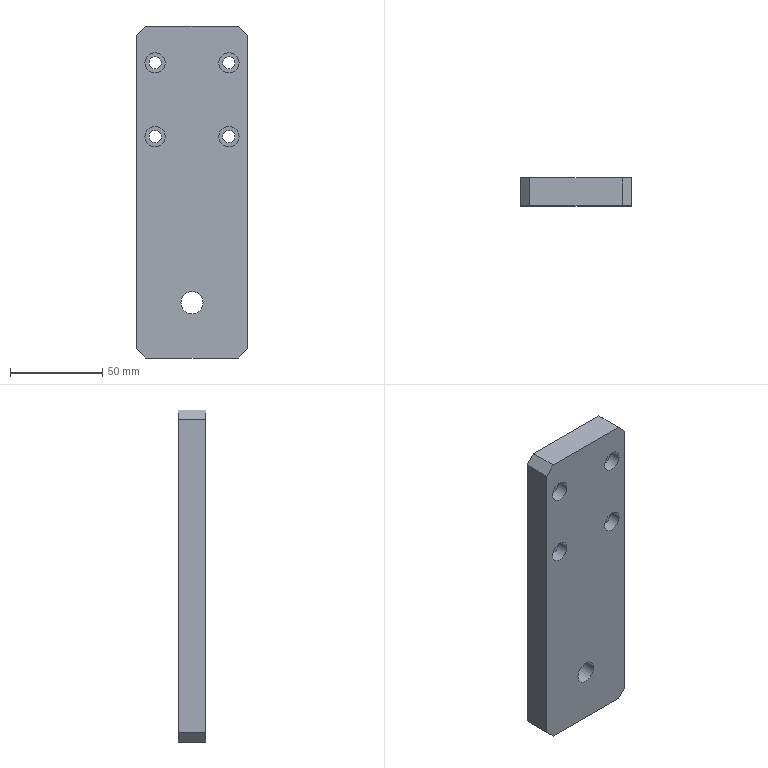Component | SolidWorks | 8TC-A15004-80-15A-5 | 1 solid | 32 faces | box 60 x 15 x 180 mm | volume 155944 mm3 | cylinder 18 | plane 14 | commonest cylinder face diameters 11 x8 6.6 x8 12 x2 | material A3
build123d program:
from build123d import *

# Parameters (mm, degrees)
SKETCH1_W                                       = 180
SKETCH1_H                                       = 60
BOSS_EXTRUDE1_DEPTH                             = 7.5
SKETCH2_R                                       = 6
CUT_EXTRUDE1_DEPTH                              = 97.047
CHAMFER1_SIZE                                   = 5
M6_HEX_SOCKET_HEAD_CAP_SCREW_CBORE1_D           = 6.6
M6_HEX_SOCKET_HEAD_CAP_SCREW_CBORE1_CBORE_D     = 11
M6_HEX_SOCKET_HEAD_CAP_SCREW_CBORE1_CBORE_DEPTH = 6.4


with BuildPart() as part:
    # Sketch1 → Boss-Extrude1 (new, symmetric)
    with BuildSketch(Plane(origin=(0, 0, 0), x_dir=(1, 0, 0), z_dir=(0, 1, 0))):
        Rectangle(SKETCH1_W, SKETCH1_H)
    extrude(amount=BOSS_EXTRUDE1_DEPTH, both=True)

    # Sketch2 → Cut-Extrude1 (cut, through all)
    with BuildSketch(Plane(origin=(0, 7.5, 0), x_dir=(1, 0, 0), z_dir=(0, 1, 0))):
        with Locations(Location((60, 0, 0), (0, 0, 270))):
            Circle(SKETCH2_R)
    extrude(amount=-CUT_EXTRUDE1_DEPTH, mode=Mode.SUBTRACT)

    # Chamfer1
    chamfer1_edges = [part.edges().sort_by_distance(p)[0] for p in [
        (90, 0, 30),
        (-90, 0, 30),
        (-90, 0, -30),
        (90, 0, -30),
    ]]
    chamfer(chamfer1_edges, length=CHAMFER1_SIZE)

    # M6 Hex Socket Head Cap Screw CBORE1 (through all)
    with Locations(Plane(origin=(0, 7.5, 0), x_dir=(1, 0, 0), z_dir=(0, 1, 0))):
        with Locations((-70, 20), (-30, 20), (-30, -20), (-70, -20)):
            CounterBoreHole(M6_HEX_SOCKET_HEAD_CAP_SCREW_CBORE1_D / 2, M6_HEX_SOCKET_HEAD_CAP_SCREW_CBORE1_CBORE_D / 2, M6_HEX_SOCKET_HEAD_CAP_SCREW_CBORE1_CBORE_DEPTH)


solid = part.part

# Placed as in the assembly
solid = solid.moved(Location((40, -15, -690), (180, -90, 0)))
STEP:
#1=CARTESIAN_POINT('',(2.579,-0.6339,-24.409));
#2=VERTEX_POINT('',#1);
#3=CARTESIAN_POINT('',(2.146,-0.6339,-24.409));
#4=VERTEX_POINT('',#3);
#5=CARTESIAN_POINT('',(2.362,-0.6339,-24.409));
#6=DIRECTION('',(0.,-1.,0.));
#7=DIRECTION('',(-1.,0.,0.));
#8=AXIS2_PLACEMENT_3D('',#5,#6,#7);
#9=CIRCLE('',#8,0.2165);
#10=EDGE_CURVE('',#2,#4,#9,.T.);
#11=ORIENTED_EDGE('',*,*,#10,.F.);
#12=CARTESIAN_POINT('',(2.579,-0.8858,-24.409));
#13=VERTEX_POINT('',#12);
#14=CARTESIAN_POINT('',(2.579,-0.8858,-24.409));
#15=DIRECTION('',(0.,-1.,0.));
#16=VECTOR('',#15,39.37);
#17=LINE('',#14,#16);
#18=EDGE_CURVE('',#2,#13,#17,.T.);
#19=ORIENTED_EDGE('',*,*,#18,.T.);
#20=CARTESIAN_POINT('',(2.146,-0.8858,-24.409));
#21=VERTEX_POINT('',#20);
#22=CARTESIAN_POINT('',(2.362,-0.8858,-24.409));
#23=DIRECTION('',(0.,-1.,0.));
#24=DIRECTION('',(-1.,0.,0.));
#25=AXIS2_PLACEMENT_3D('',#22,#23,#24);
#26=CIRCLE('',#25,0.2165);
#27=EDGE_CURVE('',#13,#21,#26,.T.);
#28=ORIENTED_EDGE('',*,*,#27,.T.);
#29=CARTESIAN_POINT('',(2.146,-0.8858,-24.409));
#30=DIRECTION('',(0.,-1.,0.));
#31=VECTOR('',#30,39.37);
#32=LINE('',#29,#31);
#33=EDGE_CURVE('',#4,#21,#32,.T.);
#34=ORIENTED_EDGE('',*,*,#33,.F.);
#35=EDGE_LOOP('',(#11,#19,#28,#34));
#36=FACE_OUTER_BOUND('',#35,.T.);
#37=CARTESIAN_POINT('',(2.362,-0.8858,-24.409));
#38=DIRECTION('',(0.,-1.,0.));
#39=DIRECTION('',(-1.,0.,0.));
#40=AXIS2_PLACEMENT_3D('',#37,#38,#39);
#41=CYLINDRICAL_SURFACE('',#40,0.2165);
#42=ADVANCED_FACE('',(#36),#41,.F.);
#43=CARTESIAN_POINT('',(2.492,-0.2953,-24.409));
#44=VERTEX_POINT('',#43);
#45=CARTESIAN_POINT('',(2.232,-0.2953,-24.409));
#46=VERTEX_POINT('',#45);
#47=CARTESIAN_POINT('',(2.362,-0.2953,-24.409));
#48=DIRECTION('',(0.,-1.,0.));
#49=DIRECTION('',(-1.,0.,0.));
#50=AXIS2_PLACEMENT_3D('',#47,#48,#49);
#51=CIRCLE('',#50,0.1299);
#52=EDGE_CURVE('',#44,#46,#51,.T.);
#53=ORIENTED_EDGE('',*,*,#52,.F.);
#54=CARTESIAN_POINT('',(2.492,-0.6339,-24.409));
#55=VERTEX_POINT('',#54);
#56=CARTESIAN_POINT('',(2.492,-0.8858,-24.409));
#57=DIRECTION('',(0.,-1.,0.));
#58=VECTOR('',#57,39.37);
#59=LINE('',#56,#58);
#60=EDGE_CURVE('',#44,#55,#59,.T.);
#61=ORIENTED_EDGE('',*,*,#60,.T.);
#62=CARTESIAN_POINT('',(2.232,-0.6339,-24.409));
#63=VERTEX_POINT('',#62);
#64=CARTESIAN_POINT('',(2.362,-0.6339,-24.409));
#65=DIRECTION('',(0.,-1.,0.));
#66=DIRECTION('',(-1.,0.,0.));
#67=AXIS2_PLACEMENT_3D('',#64,#65,#66);
#68=CIRCLE('',#67,0.1299);
#69=EDGE_CURVE('',#55,#63,#68,.T.);
#70=ORIENTED_EDGE('',*,*,#69,.T.);
#71=CARTESIAN_POINT('',(2.232,-0.8858,-24.409));
#72=DIRECTION('',(0.,-1.,0.));
#73=VECTOR('',#72,39.37);
#74=LINE('',#71,#73);
#75=EDGE_CURVE('',#46,#63,#74,.T.);
#76=ORIENTED_EDGE('',*,*,#75,.F.);
#77=EDGE_LOOP('',(#53,#61,#70,#76));
#78=FACE_OUTER_BOUND('',#77,.T.);
#79=CARTESIAN_POINT('',(2.362,-0.8858,-24.409));
#80=DIRECTION('',(0.,-1.,0.));
#81=DIRECTION('',(-1.,0.,0.));
#82=AXIS2_PLACEMENT_3D('',#79,#80,#81);
#83=CYLINDRICAL_SURFACE('',#82,0.1299);
#84=ADVANCED_FACE('',(#78),#83,.F.);
#85=CARTESIAN_POINT('',(2.579,-0.6339,-25.984));
#86=VERTEX_POINT('',#85);
#87=CARTESIAN_POINT('',(2.146,-0.6339,-25.984));
#88=VERTEX_POINT('',#87);
#89=CARTESIAN_POINT('',(2.362,-0.6339,-25.984));
#90=DIRECTION('',(0.,-1.,0.));
#91=DIRECTION('',(-1.,0.,0.));
#92=AXIS2_PLACEMENT_3D('',#89,#90,#91);
#93=CIRCLE('',#92,0.2165);
#94=EDGE_CURVE('',#86,#88,#93,.T.);
#95=ORIENTED_EDGE('',*,*,#94,.F.);
#96=CARTESIAN_POINT('',(2.579,-0.8858,-25.984));
#97=VERTEX_POINT('',#96);
#98=CARTESIAN_POINT('',(2.579,-0.8858,-25.984));
#99=DIRECTION('',(0.,-1.,0.));
#100=VECTOR('',#99,39.37);
#101=LINE('',#98,#100);
#102=EDGE_CURVE('',#86,#97,#101,.T.);
#103=ORIENTED_EDGE('',*,*,#102,.T.);
#104=CARTESIAN_POINT('',(2.146,-0.8858,-25.984));
#105=VERTEX_POINT('',#104);
#106=CARTESIAN_POINT('',(2.362,-0.8858,-25.984));
#107=DIRECTION('',(0.,-1.,0.));
#108=DIRECTION('',(-1.,0.,0.));
#109=AXIS2_PLACEMENT_3D('',#106,#107,#108);
#110=CIRCLE('',#109,0.2165);
#111=EDGE_CURVE('',#97,#105,#110,.T.);
#112=ORIENTED_EDGE('',*,*,#111,.T.);
#113=CARTESIAN_POINT('',(2.146,-0.8858,-25.984));
#114=DIRECTION('',(0.,-1.,0.));
#115=VECTOR('',#114,39.37);
#116=LINE('',#113,#115);
#117=EDGE_CURVE('',#88,#105,#116,.T.);
#118=ORIENTED_EDGE('',*,*,#117,.F.);
#119=EDGE_LOOP('',(#95,#103,#112,#118));
#120=FACE_OUTER_BOUND('',#119,.T.);
#121=CARTESIAN_POINT('',(2.362,-0.8858,-25.984));
#122=DIRECTION('',(0.,-1.,0.));
#123=DIRECTION('',(-1.,0.,0.));
#124=AXIS2_PLACEMENT_3D('',#121,#122,#123);
#125=CYLINDRICAL_SURFACE('',#124,0.2165);
#126=ADVANCED_FACE('',(#120),#125,.F.);
#127=CARTESIAN_POINT('',(2.492,-0.2953,-25.984));
#128=VERTEX_POINT('',#127);
#129=CARTESIAN_POINT('',(2.232,-0.2953,-25.984));
#130=VERTEX_POINT('',#129);
#131=CARTESIAN_POINT('',(2.362,-0.2953,-25.984));
#132=DIRECTION('',(0.,-1.,0.));
#133=DIRECTION('',(-1.,0.,0.));
#134=AXIS2_PLACEMENT_3D('',#131,#132,#133);
#135=CIRCLE('',#134,0.1299);
#136=EDGE_CURVE('',#128,#130,#135,.T.);
#137=ORIENTED_EDGE('',*,*,#136,.F.);
#138=CARTESIAN_POINT('',(2.492,-0.6339,-25.984));
#139=VERTEX_POINT('',#138);
#140=CARTESIAN_POINT('',(2.492,-0.8858,-25.984));
#141=DIRECTION('',(0.,-1.,0.));
#142=VECTOR('',#141,39.37);
#143=LINE('',#140,#142);
#144=EDGE_CURVE('',#128,#139,#143,.T.);
#145=ORIENTED_EDGE('',*,*,#144,.T.);
#146=CARTESIAN_POINT('',(2.232,-0.6339,-25.984));
#147=VERTEX_POINT('',#146);
#148=CARTESIAN_POINT('',(2.362,-0.6339,-25.984));
#149=DIRECTION('',(0.,-1.,0.));
#150=DIRECTION('',(-1.,0.,0.));
#151=AXIS2_PLACEMENT_3D('',#148,#149,#150);
#152=CIRCLE('',#151,0.1299);
#153=EDGE_CURVE('',#139,#147,#152,.T.);
#154=ORIENTED_EDGE('',*,*,#153,.T.);
#155=CARTESIAN_POINT('',(2.232,-0.8858,-25.984));
#156=DIRECTION('',(0.,-1.,0.));
#157=VECTOR('',#156,39.37);
#158=LINE('',#155,#157);
#159=EDGE_CURVE('',#130,#147,#158,.T.);
#160=ORIENTED_EDGE('',*,*,#159,.F.);
#161=EDGE_LOOP('',(#137,#145,#154,#160));
#162=FACE_OUTER_BOUND('',#161,.T.);
#163=CARTESIAN_POINT('',(2.362,-0.8858,-25.984));
#164=DIRECTION('',(0.,-1.,0.));
#165=DIRECTION('',(-1.,0.,0.));
#166=AXIS2_PLACEMENT_3D('',#163,#164,#165);
#167=CYLINDRICAL_SURFACE('',#166,0.1299);
#168=ADVANCED_FACE('',(#162),#167,.F.);
#169=CARTESIAN_POINT('',(1.004,-0.6339,-25.984));
#170=VERTEX_POINT('',#169);
#171=CARTESIAN_POINT('',(0.5709,-0.6339,-25.984));
#172=VERTEX_POINT('',#171);
#173=CARTESIAN_POINT('',(0.7874,-0.6339,-25.984));
#174=DIRECTION('',(0.,-1.,0.));
#175=DIRECTION('',(-1.,0.,0.));
#176=AXIS2_PLACEMENT_3D('',#173,#174,#175);
#177=CIRCLE('',#176,0.2165);
#178=EDGE_CURVE('',#170,#172,#177,.T.);
#179=ORIENTED_EDGE('',*,*,#178,.F.);
#180=CARTESIAN_POINT('',(1.004,-0.8858,-25.984));
#181=VERTEX_POINT('',#180);
#182=CARTESIAN_POINT('',(1.004,-0.8858,-25.984));
#183=DIRECTION('',(0.,-1.,0.));
#184=VECTOR('',#183,39.37);
#185=LINE('',#182,#184);
#186=EDGE_CURVE('',#170,#181,#185,.T.);
#187=ORIENTED_EDGE('',*,*,#186,.T.);
#188=CARTESIAN_POINT('',(0.5709,-0.8858,-25.984));
#189=VERTEX_POINT('',#188);
#190=CARTESIAN_POINT('',(0.7874,-0.8858,-25.984));
#191=DIRECTION('',(0.,-1.,0.));
#192=DIRECTION('',(-1.,0.,0.));
#193=AXIS2_PLACEMENT_3D('',#190,#191,#192);
#194=CIRCLE('',#193,0.2165);
#195=EDGE_CURVE('',#181,#189,#194,.T.);
#196=ORIENTED_EDGE('',*,*,#195,.T.);
#197=CARTESIAN_POINT('',(0.5709,-0.8858,-25.984));
#198=DIRECTION('',(0.,-1.,0.));
#199=VECTOR('',#198,39.37);
#200=LINE('',#197,#199);
#201=EDGE_CURVE('',#172,#189,#200,.T.);
#202=ORIENTED_EDGE('',*,*,#201,.F.);
#203=EDGE_LOOP('',(#179,#187,#196,#202));
#204=FACE_OUTER_BOUND('',#203,.T.);
#205=CARTESIAN_POINT('',(0.7874,-0.8858,-25.984));
#206=DIRECTION('',(0.,-1.,0.));
#207=DIRECTION('',(-1.,0.,0.));
#208=AXIS2_PLACEMENT_3D('',#205,#206,#207);
#209=CYLINDRICAL_SURFACE('',#208,0.2165);
#210=ADVANCED_FACE('',(#204),#209,.F.);
#211=CARTESIAN_POINT('',(0.9173,-0.2953,-25.984));
#212=VERTEX_POINT('',#211);
#213=CARTESIAN_POINT('',(0.6575,-0.2953,-25.984));
#214=VERTEX_POINT('',#213);
#215=CARTESIAN_POINT('',(0.7874,-0.2953,-25.984));
#216=DIRECTION('',(0.,-1.,0.));
#217=DIRECTION('',(-1.,0.,0.));
#218=AXIS2_PLACEMENT_3D('',#215,#216,#217);
#219=CIRCLE('',#218,0.1299);
#220=EDGE_CURVE('',#212,#214,#219,.T.);
#221=ORIENTED_EDGE('',*,*,#220,.F.);
#222=CARTESIAN_POINT('',(0.9173,-0.6339,-25.984));
#223=VERTEX_POINT('',#222);
#224=CARTESIAN_POINT('',(0.9173,-0.8858,-25.984));
#225=DIRECTION('',(0.,-1.,0.));
#226=VECTOR('',#225,39.37);
#227=LINE('',#224,#226);
#228=EDGE_CURVE('',#212,#223,#227,.T.);
#229=ORIENTED_EDGE('',*,*,#228,.T.);
#230=CARTESIAN_POINT('',(0.6575,-0.6339,-25.984));
#231=VERTEX_POINT('',#230);
#232=CARTESIAN_POINT('',(0.7874,-0.6339,-25.984));
#233=DIRECTION('',(0.,-1.,0.));
#234=DIRECTION('',(-1.,0.,0.));
#235=AXIS2_PLACEMENT_3D('',#232,#233,#234);
#236=CIRCLE('',#235,0.1299);
#237=EDGE_CURVE('',#223,#231,#236,.T.);
#238=ORIENTED_EDGE('',*,*,#237,.T.);
#239=CARTESIAN_POINT('',(0.6575,-0.8858,-25.984));
#240=DIRECTION('',(0.,-1.,0.));
#241=VECTOR('',#240,39.37);
#242=LINE('',#239,#241);
#243=EDGE_CURVE('',#214,#231,#242,.T.);
#244=ORIENTED_EDGE('',*,*,#243,.F.);
#245=EDGE_LOOP('',(#221,#229,#238,#244));
#246=FACE_OUTER_BOUND('',#245,.T.);
#247=CARTESIAN_POINT('',(0.7874,-0.8858,-25.984));
#248=DIRECTION('',(0.,-1.,0.));
#249=DIRECTION('',(-1.,0.,0.));
#250=AXIS2_PLACEMENT_3D('',#247,#248,#249);
#251=CYLINDRICAL_SURFACE('',#250,0.1299);
#252=ADVANCED_FACE('',(#246),#251,.F.);
#253=CARTESIAN_POINT('',(1.004,-0.6339,-24.409));
#254=VERTEX_POINT('',#253);
#255=CARTESIAN_POINT('',(0.5709,-0.6339,-24.409));
#256=VERTEX_POINT('',#255);
#257=CARTESIAN_POINT('',(0.7874,-0.6339,-24.409));
#258=DIRECTION('',(0.,-1.,0.));
#259=DIRECTION('',(-1.,0.,0.));
#260=AXIS2_PLACEMENT_3D('',#257,#258,#259);
#261=CIRCLE('',#260,0.2165);
#262=EDGE_CURVE('',#254,#256,#261,.T.);
#263=ORIENTED_EDGE('',*,*,#262,.F.);
#264=CARTESIAN_POINT('',(1.004,-0.8858,-24.409));
#265=VERTEX_POINT('',#264);
#266=CARTESIAN_POINT('',(1.004,-0.8858,-24.409));
#267=DIRECTION('',(0.,-1.,0.));
#268=VECTOR('',#267,39.37);
#269=LINE('',#266,#268);
#270=EDGE_CURVE('',#254,#265,#269,.T.);
#271=ORIENTED_EDGE('',*,*,#270,.T.);
#272=CARTESIAN_POINT('',(0.5709,-0.8858,-24.409));
#273=VERTEX_POINT('',#272);
#274=CARTESIAN_POINT('',(0.7874,-0.8858,-24.409));
#275=DIRECTION('',(0.,-1.,0.));
#276=DIRECTION('',(-1.,0.,0.));
#277=AXIS2_PLACEMENT_3D('',#274,#275,#276);
#278=CIRCLE('',#277,0.2165);
#279=EDGE_CURVE('',#265,#273,#278,.T.);
#280=ORIENTED_EDGE('',*,*,#279,.T.);
#281=CARTESIAN_POINT('',(0.5709,-0.8858,-24.409));
#282=DIRECTION('',(0.,-1.,0.));
#283=VECTOR('',#282,39.37);
#284=LINE('',#281,#283);
#285=EDGE_CURVE('',#256,#273,#284,.T.);
#286=ORIENTED_EDGE('',*,*,#285,.F.);
#287=EDGE_LOOP('',(#263,#271,#280,#286));
#288=FACE_OUTER_BOUND('',#287,.T.);
#289=CARTESIAN_POINT('',(0.7874,-0.8858,-24.409));
#290=DIRECTION('',(0.,-1.,0.));
#291=DIRECTION('',(-1.,0.,0.));
#292=AXIS2_PLACEMENT_3D('',#289,#290,#291);
#293=CYLINDRICAL_SURFACE('',#292,0.2165);
#294=ADVANCED_FACE('',(#288),#293,.F.);
#295=CARTESIAN_POINT('',(0.9173,-0.2953,-24.409));
#296=VERTEX_POINT('',#295);
#297=CARTESIAN_POINT('',(0.6575,-0.2953,-24.409));
#298=VERTEX_POINT('',#297);
#299=CARTESIAN_POINT('',(0.7874,-0.2953,-24.409));
#300=DIRECTION('',(0.,-1.,0.));
#301=DIRECTION('',(-1.,0.,0.));
#302=AXIS2_PLACEMENT_3D('',#299,#300,#301);
#303=CIRCLE('',#302,0.1299);
#304=EDGE_CURVE('',#296,#298,#303,.T.);
#305=ORIENTED_EDGE('',*,*,#304,.F.);
#306=CARTESIAN_POINT('',(0.9173,-0.6339,-24.409));
#307=VERTEX_POINT('',#306);
#308=CARTESIAN_POINT('',(0.9173,-0.8858,-24.409));
#309=DIRECTION('',(0.,-1.,0.));
#310=VECTOR('',#309,39.37);
#311=LINE('',#308,#310);
#312=EDGE_CURVE('',#296,#307,#311,.T.);
#313=ORIENTED_EDGE('',*,*,#312,.T.);
#314=CARTESIAN_POINT('',(0.6575,-0.6339,-24.409));
#315=VERTEX_POINT('',#314);
#316=CARTESIAN_POINT('',(0.7874,-0.6339,-24.409));
#317=DIRECTION('',(0.,-1.,0.));
#318=DIRECTION('',(-1.,0.,0.));
#319=AXIS2_PLACEMENT_3D('',#316,#317,#318);
#320=CIRCLE('',#319,0.1299);
#321=EDGE_CURVE('',#307,#315,#320,.T.);
#322=ORIENTED_EDGE('',*,*,#321,.T.);
#323=CARTESIAN_POINT('',(0.6575,-0.8858,-24.409));
#324=DIRECTION('',(0.,-1.,0.));
#325=VECTOR('',#324,39.37);
#326=LINE('',#323,#325);
#327=EDGE_CURVE('',#298,#315,#326,.T.);
#328=ORIENTED_EDGE('',*,*,#327,.F.);
#329=EDGE_LOOP('',(#305,#313,#322,#328));
#330=FACE_OUTER_BOUND('',#329,.T.);
#331=CARTESIAN_POINT('',(0.7874,-0.8858,-24.409));
#332=DIRECTION('',(0.,-1.,0.));
#333=DIRECTION('',(-1.,0.,0.));
#334=AXIS2_PLACEMENT_3D('',#331,#332,#333);
#335=CYLINDRICAL_SURFACE('',#334,0.1299);
#336=ADVANCED_FACE('',(#330),#335,.F.);
#337=CARTESIAN_POINT('',(1.811,-0.2953,-29.528));
#338=VERTEX_POINT('',#337);
#339=CARTESIAN_POINT('',(1.339,-0.2953,-29.528));
#340=VERTEX_POINT('',#339);
#341=CARTESIAN_POINT('',(1.575,-0.2953,-29.528));
#342=DIRECTION('',(0.,-1.,0.));
#343=DIRECTION('',(-1.,0.,0.));
#344=AXIS2_PLACEMENT_3D('',#341,#342,#343);
#345=CIRCLE('',#344,0.2362);
#346=EDGE_CURVE('',#338,#340,#345,.T.);
#347=ORIENTED_EDGE('',*,*,#346,.F.);
#348=CARTESIAN_POINT('',(1.811,-0.8858,-29.528));
#349=VERTEX_POINT('',#348);
#350=CARTESIAN_POINT('',(1.811,-0.2953,-29.528));
#351=DIRECTION('',(0.,-1.,0.));
#352=VECTOR('',#351,39.37);
#353=LINE('',#350,#352);
#354=EDGE_CURVE('',#338,#349,#353,.T.);
#355=ORIENTED_EDGE('',*,*,#354,.T.);
#356=CARTESIAN_POINT('',(1.339,-0.8858,-29.528));
#357=VERTEX_POINT('',#356);
#358=CARTESIAN_POINT('',(1.575,-0.8858,-29.528));
#359=DIRECTION('',(0.,-1.,0.));
#360=DIRECTION('',(-1.,0.,0.));
#361=AXIS2_PLACEMENT_3D('',#358,#359,#360);
#362=CIRCLE('',#361,0.2362);
#363=EDGE_CURVE('',#349,#357,#362,.T.);
#364=ORIENTED_EDGE('',*,*,#363,.T.);
#365=CARTESIAN_POINT('',(1.339,-0.2953,-29.528));
#366=DIRECTION('',(0.,-1.,0.));
#367=VECTOR('',#366,39.37);
#368=LINE('',#365,#367);
#369=EDGE_CURVE('',#340,#357,#368,.T.);
#370=ORIENTED_EDGE('',*,*,#369,.F.);
#371=EDGE_LOOP('',(#347,#355,#364,#370));
#372=FACE_OUTER_BOUND('',#371,.T.);
#373=CARTESIAN_POINT('',(1.575,-0.2953,-29.528));
#374=DIRECTION('',(0.,-1.,0.));
#375=DIRECTION('',(-1.,0.,0.));
#376=AXIS2_PLACEMENT_3D('',#373,#374,#375);
#377=CYLINDRICAL_SURFACE('',#376,0.2362);
#378=ADVANCED_FACE('',(#372),#377,.F.);
#379=CARTESIAN_POINT('',(0.5906,-0.8858,-30.709));
#380=VERTEX_POINT('',#379);
#381=CARTESIAN_POINT('',(2.559,-0.8858,-30.709));
#382=VERTEX_POINT('',#381);
#383=CARTESIAN_POINT('',(0.3937,-0.8858,-30.709));
#384=DIRECTION('',(1.,0.,-0.));
#385=VECTOR('',#384,39.37);
#386=LINE('',#383,#385);
#387=EDGE_CURVE('',#380,#382,#386,.T.);
#388=ORIENTED_EDGE('',*,*,#387,.F.);
#389=CARTESIAN_POINT('',(0.5906,-0.2953,-30.709));
#390=VERTEX_POINT('',#389);
#391=CARTESIAN_POINT('',(0.5906,-0.8858,-30.709));
#392=DIRECTION('',(0.,1.,0.));
#393=VECTOR('',#392,39.37);
#394=LINE('',#391,#393);
#395=EDGE_CURVE('',#380,#390,#394,.T.);
#396=ORIENTED_EDGE('',*,*,#395,.T.);
#397=CARTESIAN_POINT('',(2.559,-0.2953,-30.709));
#398=VERTEX_POINT('',#397);
#399=CARTESIAN_POINT('',(0.3937,-0.2953,-30.709));
#400=DIRECTION('',(1.,0.,-0.));
#401=VECTOR('',#400,39.37);
#402=LINE('',#399,#401);
#403=EDGE_CURVE('',#390,#398,#402,.T.);
#404=ORIENTED_EDGE('',*,*,#403,.T.);
#405=CARTESIAN_POINT('',(2.559,-0.8858,-30.709));
#406=DIRECTION('',(0.,-1.,0.));
#407=VECTOR('',#406,39.37);
#408=LINE('',#405,#407);
#409=EDGE_CURVE('',#398,#382,#408,.T.);
#410=ORIENTED_EDGE('',*,*,#409,.T.);
#411=EDGE_LOOP('',(#388,#396,#404,#410));
#412=FACE_OUTER_BOUND('',#411,.T.);
#413=CARTESIAN_POINT('',(0.3937,-0.8858,-30.709));
#414=DIRECTION('',(0.,0.,1.));
#415=DIRECTION('',(-1.,0.,0.));
#416=AXIS2_PLACEMENT_3D('',#413,#414,#415);
#417=PLANE('',#416);
#418=ADVANCED_FACE('',(#412),#417,.F.);
#419=CARTESIAN_POINT('',(2.756,-0.2953,-30.512));
#420=VERTEX_POINT('',#419);
#421=CARTESIAN_POINT('',(2.756,-0.2953,-23.819));
#422=VERTEX_POINT('',#421);
#423=CARTESIAN_POINT('',(2.756,-0.2953,-23.622));
#424=DIRECTION('',(0.,0.,1.));
#425=VECTOR('',#424,39.37);
#426=LINE('',#423,#425);
#427=EDGE_CURVE('',#420,#422,#426,.T.);
#428=ORIENTED_EDGE('',*,*,#427,.T.);
#429=CARTESIAN_POINT('',(2.756,-0.8858,-23.819));
#430=VERTEX_POINT('',#429);
#431=CARTESIAN_POINT('',(2.756,-0.8858,-23.819));
#432=DIRECTION('',(0.,-1.,0.));
#433=VECTOR('',#432,39.37);
#434=LINE('',#431,#433);
#435=EDGE_CURVE('',#422,#430,#434,.T.);
#436=ORIENTED_EDGE('',*,*,#435,.T.);
#437=CARTESIAN_POINT('',(2.756,-0.8858,-30.512));
#438=VERTEX_POINT('',#437);
#439=CARTESIAN_POINT('',(2.756,-0.8858,-23.622));
#440=DIRECTION('',(0.,0.,1.));
#441=VECTOR('',#440,39.37);
#442=LINE('',#439,#441);
#443=EDGE_CURVE('',#438,#430,#442,.T.);
#444=ORIENTED_EDGE('',*,*,#443,.F.);
#445=CARTESIAN_POINT('',(2.756,-0.8858,-30.512));
#446=DIRECTION('',(0.,1.,0.));
#447=VECTOR('',#446,39.37);
#448=LINE('',#445,#447);
#449=EDGE_CURVE('',#438,#420,#448,.T.);
#450=ORIENTED_EDGE('',*,*,#449,.T.);
#451=EDGE_LOOP('',(#428,#436,#444,#450));
#452=FACE_OUTER_BOUND('',#451,.T.);
#453=CARTESIAN_POINT('',(2.756,-0.8858,-23.622));
#454=DIRECTION('',(-1.,0.,0.));
#455=DIRECTION('',(-0.,0.,-1.));
#456=AXIS2_PLACEMENT_3D('',#453,#454,#455);
#457=PLANE('',#456);
#458=ADVANCED_FACE('',(#452),#457,.F.);
#459=CARTESIAN_POINT('',(2.559,-0.2953,-23.622));
#460=VERTEX_POINT('',#459);
#461=CARTESIAN_POINT('',(0.5906,-0.2953,-23.622));
#462=VERTEX_POINT('',#461);
#463=CARTESIAN_POINT('',(0.3937,-0.2953,-23.622));
#464=DIRECTION('',(-1.,0.,0.));
#465=VECTOR('',#464,39.37);
#466=LINE('',#463,#465);
#467=EDGE_CURVE('',#460,#462,#466,.T.);
#468=ORIENTED_EDGE('',*,*,#467,.T.);
#469=CARTESIAN_POINT('',(0.5906,-0.8858,-23.622));
#470=VERTEX_POINT('',#469);
#471=CARTESIAN_POINT('',(0.5906,-0.8858,-23.622));
#472=DIRECTION('',(0.,-1.,0.));
#473=VECTOR('',#472,39.37);
#474=LINE('',#471,#473);
#475=EDGE_CURVE('',#462,#470,#474,.T.);
#476=ORIENTED_EDGE('',*,*,#475,.T.);
#477=CARTESIAN_POINT('',(2.559,-0.8858,-23.622));
#478=VERTEX_POINT('',#477);
#479=CARTESIAN_POINT('',(0.3937,-0.8858,-23.622));
#480=DIRECTION('',(-1.,0.,0.));
#481=VECTOR('',#480,39.37);
#482=LINE('',#479,#481);
#483=EDGE_CURVE('',#478,#470,#482,.T.);
#484=ORIENTED_EDGE('',*,*,#483,.F.);
#485=CARTESIAN_POINT('',(2.559,-0.8858,-23.622));
#486=DIRECTION('',(0.,1.,0.));
#487=VECTOR('',#486,39.37);
#488=LINE('',#485,#487);
#489=EDGE_CURVE('',#478,#460,#488,.T.);
#490=ORIENTED_EDGE('',*,*,#489,.T.);
#491=EDGE_LOOP('',(#468,#476,#484,#490));
#492=FACE_OUTER_BOUND('',#491,.T.);
#493=CARTESIAN_POINT('',(0.3937,-0.8858,-23.622));
#494=DIRECTION('',(-0.,0.,-1.));
#495=DIRECTION('',(1.,0.,-0.));
#496=AXIS2_PLACEMENT_3D('',#493,#494,#495);
#497=PLANE('',#496);
#498=ADVANCED_FACE('',(#492),#497,.F.);
#499=CARTESIAN_POINT('',(0.3937,-0.8858,-23.819));
#500=VERTEX_POINT('',#499);
#501=CARTESIAN_POINT('',(0.3937,-0.8858,-30.512));
#502=VERTEX_POINT('',#501);
#503=CARTESIAN_POINT('',(0.3937,-0.8858,-23.622));
#504=DIRECTION('',(-0.,0.,-1.));
#505=VECTOR('',#504,39.37);
#506=LINE('',#503,#505);
#507=EDGE_CURVE('',#500,#502,#506,.T.);
#508=ORIENTED_EDGE('',*,*,#507,.F.);
#509=CARTESIAN_POINT('',(0.3937,-0.2953,-23.819));
#510=VERTEX_POINT('',#509);
#511=CARTESIAN_POINT('',(0.3937,-0.8858,-23.819));
#512=DIRECTION('',(0.,1.,0.));
#513=VECTOR('',#512,39.37);
#514=LINE('',#511,#513);
#515=EDGE_CURVE('',#500,#510,#514,.T.);
#516=ORIENTED_EDGE('',*,*,#515,.T.);
#517=CARTESIAN_POINT('',(0.3937,-0.2953,-30.512));
#518=VERTEX_POINT('',#517);
#519=CARTESIAN_POINT('',(0.3937,-0.2953,-23.622));
#520=DIRECTION('',(-0.,0.,-1.));
#521=VECTOR('',#520,39.37);
#522=LINE('',#519,#521);
#523=EDGE_CURVE('',#510,#518,#522,.T.);
#524=ORIENTED_EDGE('',*,*,#523,.T.);
#525=CARTESIAN_POINT('',(0.3937,-0.8858,-30.512));
#526=DIRECTION('',(0.,-1.,0.));
#527=VECTOR('',#526,39.37);
#528=LINE('',#525,#527);
#529=EDGE_CURVE('',#518,#502,#528,.T.);
#530=ORIENTED_EDGE('',*,*,#529,.T.);
#531=EDGE_LOOP('',(#508,#516,#524,#530));
#532=FACE_OUTER_BOUND('',#531,.T.);
#533=CARTESIAN_POINT('',(0.3937,-0.8858,-23.622));
#534=DIRECTION('',(1.,0.,-0.));
#535=DIRECTION('',(0.,0.,1.));
#536=AXIS2_PLACEMENT_3D('',#533,#534,#535);
#537=PLANE('',#536);
#538=ADVANCED_FACE('',(#532),#537,.F.);
#539=CARTESIAN_POINT('',(2.362,-0.8858,-24.409));
#540=DIRECTION('',(0.,-1.,0.));
#541=DIRECTION('',(-1.,0.,0.));
#542=AXIS2_PLACEMENT_3D('',#539,#540,#541);
#543=CIRCLE('',#542,0.2165);
#544=EDGE_CURVE('',#21,#13,#543,.T.);
#545=ORIENTED_EDGE('',*,*,#544,.F.);
#546=ORIENTED_EDGE('',*,*,#27,.F.);
#547=EDGE_LOOP('',(#545,#546));
#548=FACE_BOUND('',#547,.T.);
#549=CARTESIAN_POINT('',(2.362,-0.8858,-25.984));
#550=DIRECTION('',(0.,-1.,0.));
#551=DIRECTION('',(-1.,0.,0.));
#552=AXIS2_PLACEMENT_3D('',#549,#550,#551);
#553=CIRCLE('',#552,0.2165);
#554=EDGE_CURVE('',#105,#97,#553,.T.);
#555=ORIENTED_EDGE('',*,*,#554,.F.);
#556=ORIENTED_EDGE('',*,*,#111,.F.);
#557=EDGE_LOOP('',(#555,#556));
#558=FACE_BOUND('',#557,.T.);
#559=CARTESIAN_POINT('',(0.7874,-0.8858,-25.984));
#560=DIRECTION('',(0.,-1.,0.));
#561=DIRECTION('',(-1.,0.,0.));
#562=AXIS2_PLACEMENT_3D('',#559,#560,#561);
#563=CIRCLE('',#562,0.2165);
#564=EDGE_CURVE('',#189,#181,#563,.T.);
#565=ORIENTED_EDGE('',*,*,#564,.F.);
#566=ORIENTED_EDGE('',*,*,#195,.F.);
#567=EDGE_LOOP('',(#565,#566));
#568=FACE_BOUND('',#567,.T.);
#569=CARTESIAN_POINT('',(0.7874,-0.8858,-24.409));
#570=DIRECTION('',(0.,-1.,0.));
#571=DIRECTION('',(-1.,0.,0.));
#572=AXIS2_PLACEMENT_3D('',#569,#570,#571);
#573=CIRCLE('',#572,0.2165);
#574=EDGE_CURVE('',#273,#265,#573,.T.);
#575=ORIENTED_EDGE('',*,*,#574,.F.);
#576=ORIENTED_EDGE('',*,*,#279,.F.);
#577=EDGE_LOOP('',(#575,#576));
#578=FACE_BOUND('',#577,.T.);
#579=CARTESIAN_POINT('',(1.575,-0.8858,-29.528));
#580=DIRECTION('',(0.,-1.,0.));
#581=DIRECTION('',(-1.,0.,0.));
#582=AXIS2_PLACEMENT_3D('',#579,#580,#581);
#583=CIRCLE('',#582,0.2362);
#584=EDGE_CURVE('',#357,#349,#583,.T.);
#585=ORIENTED_EDGE('',*,*,#584,.F.);
#586=ORIENTED_EDGE('',*,*,#363,.F.);
#587=EDGE_LOOP('',(#585,#586));
#588=FACE_BOUND('',#587,.T.);
#589=ORIENTED_EDGE('',*,*,#483,.T.);
#590=CARTESIAN_POINT('',(0.3937,-0.8858,-23.819));
#591=DIRECTION('',(-0.7071,0.,-0.7071));
#592=VECTOR('',#591,39.37);
#593=LINE('',#590,#592);
#594=EDGE_CURVE('',#470,#500,#593,.T.);
#595=ORIENTED_EDGE('',*,*,#594,.T.);
#596=ORIENTED_EDGE('',*,*,#507,.T.);
#597=CARTESIAN_POINT('',(0.5906,-0.8858,-30.709));
#598=DIRECTION('',(0.7071,0.,-0.7071));
#599=VECTOR('',#598,39.37);
#600=LINE('',#597,#599);
#601=EDGE_CURVE('',#502,#380,#600,.T.);
#602=ORIENTED_EDGE('',*,*,#601,.T.);
#603=ORIENTED_EDGE('',*,*,#387,.T.);
#604=CARTESIAN_POINT('',(2.756,-0.8858,-30.512));
#605=DIRECTION('',(0.7071,0.,0.7071));
#606=VECTOR('',#605,39.37);
#607=LINE('',#604,#606);
#608=EDGE_CURVE('',#382,#438,#607,.T.);
#609=ORIENTED_EDGE('',*,*,#608,.T.);
#610=ORIENTED_EDGE('',*,*,#443,.T.);
#611=CARTESIAN_POINT('',(2.559,-0.8858,-23.622));
#612=DIRECTION('',(-0.7071,0.,0.7071));
#613=VECTOR('',#612,39.37);
#614=LINE('',#611,#613);
#615=EDGE_CURVE('',#430,#478,#614,.T.);
#616=ORIENTED_EDGE('',*,*,#615,.T.);
#617=EDGE_LOOP('',(#589,#595,#596,#602,#603,#609,#610,#616));
#618=FACE_OUTER_BOUND('',#617,.T.);
#619=CARTESIAN_POINT('',(1.575,-0.8858,-27.165));
#620=DIRECTION('',(0.,1.,0.));
#621=DIRECTION('',(1.,0.,-0.));
#622=AXIS2_PLACEMENT_3D('',#619,#620,#621);
#623=PLANE('',#622);
#624=ADVANCED_FACE('',(#548,#558,#568,#578,#588,#618),#623,.F.);
#625=CARTESIAN_POINT('',(2.362,-0.2953,-24.409));
#626=DIRECTION('',(0.,-1.,0.));
#627=DIRECTION('',(-1.,0.,0.));
#628=AXIS2_PLACEMENT_3D('',#625,#626,#627);
#629=CIRCLE('',#628,0.1299);
#630=EDGE_CURVE('',#46,#44,#629,.T.);
#631=ORIENTED_EDGE('',*,*,#630,.T.);
#632=ORIENTED_EDGE('',*,*,#52,.T.);
#633=EDGE_LOOP('',(#631,#632));
#634=FACE_BOUND('',#633,.T.);
#635=CARTESIAN_POINT('',(2.362,-0.2953,-25.984));
#636=DIRECTION('',(0.,-1.,0.));
#637=DIRECTION('',(-1.,0.,0.));
#638=AXIS2_PLACEMENT_3D('',#635,#636,#637);
#639=CIRCLE('',#638,0.1299);
#640=EDGE_CURVE('',#130,#128,#639,.T.);
#641=ORIENTED_EDGE('',*,*,#640,.T.);
#642=ORIENTED_EDGE('',*,*,#136,.T.);
#643=EDGE_LOOP('',(#641,#642));
#644=FACE_BOUND('',#643,.T.);
#645=CARTESIAN_POINT('',(0.7874,-0.2953,-25.984));
#646=DIRECTION('',(0.,-1.,0.));
#647=DIRECTION('',(-1.,0.,0.));
#648=AXIS2_PLACEMENT_3D('',#645,#646,#647);
#649=CIRCLE('',#648,0.1299);
#650=EDGE_CURVE('',#214,#212,#649,.T.);
#651=ORIENTED_EDGE('',*,*,#650,.T.);
#652=ORIENTED_EDGE('',*,*,#220,.T.);
#653=EDGE_LOOP('',(#651,#652));
#654=FACE_BOUND('',#653,.T.);
#655=CARTESIAN_POINT('',(0.7874,-0.2953,-24.409));
#656=DIRECTION('',(0.,-1.,0.));
#657=DIRECTION('',(-1.,0.,0.));
#658=AXIS2_PLACEMENT_3D('',#655,#656,#657);
#659=CIRCLE('',#658,0.1299);
#660=EDGE_CURVE('',#298,#296,#659,.T.);
#661=ORIENTED_EDGE('',*,*,#660,.T.);
#662=ORIENTED_EDGE('',*,*,#304,.T.);
#663=EDGE_LOOP('',(#661,#662));
#664=FACE_BOUND('',#663,.T.);
#665=CARTESIAN_POINT('',(1.575,-0.2953,-29.528));
#666=DIRECTION('',(0.,-1.,0.));
#667=DIRECTION('',(-1.,0.,0.));
#668=AXIS2_PLACEMENT_3D('',#665,#666,#667);
#669=CIRCLE('',#668,0.2362);
#670=EDGE_CURVE('',#340,#338,#669,.T.);
#671=ORIENTED_EDGE('',*,*,#670,.T.);
#672=ORIENTED_EDGE('',*,*,#346,.T.);
#673=EDGE_LOOP('',(#671,#672));
#674=FACE_BOUND('',#673,.T.);
#675=ORIENTED_EDGE('',*,*,#523,.F.);
#676=CARTESIAN_POINT('',(-0.689,-0.2953,-24.902));
#677=DIRECTION('',(0.7071,0.,0.7071));
#678=VECTOR('',#677,39.37);
#679=LINE('',#676,#678);
#680=EDGE_CURVE('',#510,#462,#679,.T.);
#681=ORIENTED_EDGE('',*,*,#680,.T.);
#682=ORIENTED_EDGE('',*,*,#467,.F.);
#683=CARTESIAN_POINT('',(3.839,-0.2953,-24.902));
#684=DIRECTION('',(0.7071,0.,-0.7071));
#685=VECTOR('',#684,39.37);
#686=LINE('',#683,#685);
#687=EDGE_CURVE('',#460,#422,#686,.T.);
#688=ORIENTED_EDGE('',*,*,#687,.T.);
#689=ORIENTED_EDGE('',*,*,#427,.F.);
#690=CARTESIAN_POINT('',(3.839,-0.2953,-29.429));
#691=DIRECTION('',(-0.7071,0.,-0.7071));
#692=VECTOR('',#691,39.37);
#693=LINE('',#690,#692);
#694=EDGE_CURVE('',#420,#398,#693,.T.);
#695=ORIENTED_EDGE('',*,*,#694,.T.);
#696=ORIENTED_EDGE('',*,*,#403,.F.);
#697=CARTESIAN_POINT('',(-0.689,-0.2953,-29.429));
#698=DIRECTION('',(-0.7071,0.,0.7071));
#699=VECTOR('',#698,39.37);
#700=LINE('',#697,#699);
#701=EDGE_CURVE('',#390,#518,#700,.T.);
#702=ORIENTED_EDGE('',*,*,#701,.T.);
#703=EDGE_LOOP('',(#675,#681,#682,#688,#689,#695,#696,#702));
#704=FACE_OUTER_BOUND('',#703,.T.);
#705=CARTESIAN_POINT('',(1.575,-0.2953,-27.165));
#706=DIRECTION('',(0.,1.,0.));
#707=DIRECTION('',(1.,0.,-0.));
#708=AXIS2_PLACEMENT_3D('',#705,#706,#707);
#709=PLANE('',#708);
#710=ADVANCED_FACE('',(#634,#644,#654,#664,#674,#704),#709,.T.);
#711=ORIENTED_EDGE('',*,*,#354,.F.);
#712=ORIENTED_EDGE('',*,*,#670,.F.);
#713=ORIENTED_EDGE('',*,*,#369,.T.);
#714=ORIENTED_EDGE('',*,*,#584,.T.);
#715=EDGE_LOOP('',(#711,#712,#713,#714));
#716=FACE_OUTER_BOUND('',#715,.T.);
#717=CARTESIAN_POINT('',(1.575,-0.2953,-29.528));
#718=DIRECTION('',(0.,-1.,0.));
#719=DIRECTION('',(-1.,0.,0.));
#720=AXIS2_PLACEMENT_3D('',#717,#718,#719);
#721=CYLINDRICAL_SURFACE('',#720,0.2362);
#722=ADVANCED_FACE('',(#716),#721,.F.);
#723=ORIENTED_EDGE('',*,*,#594,.F.);
#724=ORIENTED_EDGE('',*,*,#475,.F.);
#725=ORIENTED_EDGE('',*,*,#680,.F.);
#726=ORIENTED_EDGE('',*,*,#515,.F.);
#727=EDGE_LOOP('',(#723,#724,#725,#726));
#728=FACE_OUTER_BOUND('',#727,.T.);
#729=CARTESIAN_POINT('',(0.3937,-0.8858,-23.819));
#730=DIRECTION('',(0.7071,0.,-0.7071));
#731=DIRECTION('',(0.,1.,0.));
#732=AXIS2_PLACEMENT_3D('',#729,#730,#731);
#733=PLANE('',#732);
#734=ADVANCED_FACE('',(#728),#733,.F.);
#735=ORIENTED_EDGE('',*,*,#615,.F.);
#736=ORIENTED_EDGE('',*,*,#435,.F.);
#737=ORIENTED_EDGE('',*,*,#687,.F.);
#738=ORIENTED_EDGE('',*,*,#489,.F.);
#739=EDGE_LOOP('',(#735,#736,#737,#738));
#740=FACE_OUTER_BOUND('',#739,.T.);
#741=CARTESIAN_POINT('',(2.559,-0.8858,-23.622));
#742=DIRECTION('',(-0.7071,0.,-0.7071));
#743=DIRECTION('',(0.,1.,0.));
#744=AXIS2_PLACEMENT_3D('',#741,#742,#743);
#745=PLANE('',#744);
#746=ADVANCED_FACE('',(#740),#745,.F.);
#747=ORIENTED_EDGE('',*,*,#601,.F.);
#748=ORIENTED_EDGE('',*,*,#529,.F.);
#749=ORIENTED_EDGE('',*,*,#701,.F.);
#750=ORIENTED_EDGE('',*,*,#395,.F.);
#751=EDGE_LOOP('',(#747,#748,#749,#750));
#752=FACE_OUTER_BOUND('',#751,.T.);
#753=CARTESIAN_POINT('',(0.5906,-0.8858,-30.709));
#754=DIRECTION('',(0.7071,0.,0.7071));
#755=DIRECTION('',(0.,1.,0.));
#756=AXIS2_PLACEMENT_3D('',#753,#754,#755);
#757=PLANE('',#756);
#758=ADVANCED_FACE('',(#752),#757,.F.);
#759=ORIENTED_EDGE('',*,*,#608,.F.);
#760=ORIENTED_EDGE('',*,*,#409,.F.);
#761=ORIENTED_EDGE('',*,*,#694,.F.);
#762=ORIENTED_EDGE('',*,*,#449,.F.);
#763=EDGE_LOOP('',(#759,#760,#761,#762));
#764=FACE_OUTER_BOUND('',#763,.T.);
#765=CARTESIAN_POINT('',(2.756,-0.8858,-30.512));
#766=DIRECTION('',(-0.7071,0.,0.7071));
#767=DIRECTION('',(0.,1.,0.));
#768=AXIS2_PLACEMENT_3D('',#765,#766,#767);
#769=PLANE('',#768);
#770=ADVANCED_FACE('',(#764),#769,.F.);
#771=ORIENTED_EDGE('',*,*,#312,.F.);
#772=ORIENTED_EDGE('',*,*,#660,.F.);
#773=ORIENTED_EDGE('',*,*,#327,.T.);
#774=CARTESIAN_POINT('',(0.7874,-0.6339,-24.409));
#775=DIRECTION('',(0.,-1.,0.));
#776=DIRECTION('',(-1.,0.,0.));
#777=AXIS2_PLACEMENT_3D('',#774,#775,#776);
#778=CIRCLE('',#777,0.1299);
#779=EDGE_CURVE('',#315,#307,#778,.T.);
#780=ORIENTED_EDGE('',*,*,#779,.T.);
#781=EDGE_LOOP('',(#771,#772,#773,#780));
#782=FACE_OUTER_BOUND('',#781,.T.);
#783=CARTESIAN_POINT('',(0.7874,-0.8858,-24.409));
#784=DIRECTION('',(0.,-1.,0.));
#785=DIRECTION('',(-1.,0.,0.));
#786=AXIS2_PLACEMENT_3D('',#783,#784,#785);
#787=CYLINDRICAL_SURFACE('',#786,0.1299);
#788=ADVANCED_FACE('',(#782),#787,.F.);
#789=ORIENTED_EDGE('',*,*,#779,.F.);
#790=ORIENTED_EDGE('',*,*,#321,.F.);
#791=EDGE_LOOP('',(#789,#790));
#792=FACE_BOUND('',#791,.T.);
#793=CARTESIAN_POINT('',(0.7874,-0.6339,-24.409));
#794=DIRECTION('',(0.,-1.,0.));
#795=DIRECTION('',(-1.,0.,0.));
#796=AXIS2_PLACEMENT_3D('',#793,#794,#795);
#797=CIRCLE('',#796,0.2165);
#798=EDGE_CURVE('',#256,#254,#797,.T.);
#799=ORIENTED_EDGE('',*,*,#798,.T.);
#800=ORIENTED_EDGE('',*,*,#262,.T.);
#801=EDGE_LOOP('',(#799,#800));
#802=FACE_OUTER_BOUND('',#801,.T.);
#803=CARTESIAN_POINT('',(0.7874,-0.6339,-24.539));
#804=DIRECTION('',(0.,1.,0.));
#805=DIRECTION('',(1.,0.,-0.));
#806=AXIS2_PLACEMENT_3D('',#803,#804,#805);
#807=PLANE('',#806);
#808=ADVANCED_FACE('',(#792,#802),#807,.F.);
#809=ORIENTED_EDGE('',*,*,#270,.F.);
#810=ORIENTED_EDGE('',*,*,#798,.F.);
#811=ORIENTED_EDGE('',*,*,#285,.T.);
#812=ORIENTED_EDGE('',*,*,#574,.T.);
#813=EDGE_LOOP('',(#809,#810,#811,#812));
#814=FACE_OUTER_BOUND('',#813,.T.);
#815=CARTESIAN_POINT('',(0.7874,-0.8858,-24.409));
#816=DIRECTION('',(0.,-1.,0.));
#817=DIRECTION('',(-1.,0.,0.));
#818=AXIS2_PLACEMENT_3D('',#815,#816,#817);
#819=CYLINDRICAL_SURFACE('',#818,0.2165);
#820=ADVANCED_FACE('',(#814),#819,.F.);
#821=ORIENTED_EDGE('',*,*,#228,.F.);
#822=ORIENTED_EDGE('',*,*,#650,.F.);
#823=ORIENTED_EDGE('',*,*,#243,.T.);
#824=CARTESIAN_POINT('',(0.7874,-0.6339,-25.984));
#825=DIRECTION('',(0.,-1.,0.));
#826=DIRECTION('',(-1.,0.,0.));
#827=AXIS2_PLACEMENT_3D('',#824,#825,#826);
#828=CIRCLE('',#827,0.1299);
#829=EDGE_CURVE('',#231,#223,#828,.T.);
#830=ORIENTED_EDGE('',*,*,#829,.T.);
#831=EDGE_LOOP('',(#821,#822,#823,#830));
#832=FACE_OUTER_BOUND('',#831,.T.);
#833=CARTESIAN_POINT('',(0.7874,-0.8858,-25.984));
#834=DIRECTION('',(0.,-1.,0.));
#835=DIRECTION('',(-1.,0.,0.));
#836=AXIS2_PLACEMENT_3D('',#833,#834,#835);
#837=CYLINDRICAL_SURFACE('',#836,0.1299);
#838=ADVANCED_FACE('',(#832),#837,.F.);
#839=ORIENTED_EDGE('',*,*,#829,.F.);
#840=ORIENTED_EDGE('',*,*,#237,.F.);
#841=EDGE_LOOP('',(#839,#840));
#842=FACE_BOUND('',#841,.T.);
#843=CARTESIAN_POINT('',(0.7874,-0.6339,-25.984));
#844=DIRECTION('',(0.,-1.,0.));
#845=DIRECTION('',(-1.,0.,0.));
#846=AXIS2_PLACEMENT_3D('',#843,#844,#845);
#847=CIRCLE('',#846,0.2165);
#848=EDGE_CURVE('',#172,#170,#847,.T.);
#849=ORIENTED_EDGE('',*,*,#848,.T.);
#850=ORIENTED_EDGE('',*,*,#178,.T.);
#851=EDGE_LOOP('',(#849,#850));
#852=FACE_OUTER_BOUND('',#851,.T.);
#853=CARTESIAN_POINT('',(0.7874,-0.6339,-26.114));
#854=DIRECTION('',(0.,1.,0.));
#855=DIRECTION('',(1.,0.,-0.));
#856=AXIS2_PLACEMENT_3D('',#853,#854,#855);
#857=PLANE('',#856);
#858=ADVANCED_FACE('',(#842,#852),#857,.F.);
#859=ORIENTED_EDGE('',*,*,#186,.F.);
#860=ORIENTED_EDGE('',*,*,#848,.F.);
#861=ORIENTED_EDGE('',*,*,#201,.T.);
#862=ORIENTED_EDGE('',*,*,#564,.T.);
#863=EDGE_LOOP('',(#859,#860,#861,#862));
#864=FACE_OUTER_BOUND('',#863,.T.);
#865=CARTESIAN_POINT('',(0.7874,-0.8858,-25.984));
#866=DIRECTION('',(0.,-1.,0.));
#867=DIRECTION('',(-1.,0.,0.));
#868=AXIS2_PLACEMENT_3D('',#865,#866,#867);
#869=CYLINDRICAL_SURFACE('',#868,0.2165);
#870=ADVANCED_FACE('',(#864),#869,.F.);
#871=ORIENTED_EDGE('',*,*,#144,.F.);
#872=ORIENTED_EDGE('',*,*,#640,.F.);
#873=ORIENTED_EDGE('',*,*,#159,.T.);
#874=CARTESIAN_POINT('',(2.362,-0.6339,-25.984));
#875=DIRECTION('',(0.,-1.,0.));
#876=DIRECTION('',(-1.,0.,0.));
#877=AXIS2_PLACEMENT_3D('',#874,#875,#876);
#878=CIRCLE('',#877,0.1299);
#879=EDGE_CURVE('',#147,#139,#878,.T.);
#880=ORIENTED_EDGE('',*,*,#879,.T.);
#881=EDGE_LOOP('',(#871,#872,#873,#880));
#882=FACE_OUTER_BOUND('',#881,.T.);
#883=CARTESIAN_POINT('',(2.362,-0.8858,-25.984));
#884=DIRECTION('',(0.,-1.,0.));
#885=DIRECTION('',(-1.,0.,0.));
#886=AXIS2_PLACEMENT_3D('',#883,#884,#885);
#887=CYLINDRICAL_SURFACE('',#886,0.1299);
#888=ADVANCED_FACE('',(#882),#887,.F.);
#889=ORIENTED_EDGE('',*,*,#879,.F.);
#890=ORIENTED_EDGE('',*,*,#153,.F.);
#891=EDGE_LOOP('',(#889,#890));
#892=FACE_BOUND('',#891,.T.);
#893=CARTESIAN_POINT('',(2.362,-0.6339,-25.984));
#894=DIRECTION('',(0.,-1.,0.));
#895=DIRECTION('',(-1.,0.,0.));
#896=AXIS2_PLACEMENT_3D('',#893,#894,#895);
#897=CIRCLE('',#896,0.2165);
#898=EDGE_CURVE('',#88,#86,#897,.T.);
#899=ORIENTED_EDGE('',*,*,#898,.T.);
#900=ORIENTED_EDGE('',*,*,#94,.T.);
#901=EDGE_LOOP('',(#899,#900));
#902=FACE_OUTER_BOUND('',#901,.T.);
#903=CARTESIAN_POINT('',(2.362,-0.6339,-26.114));
#904=DIRECTION('',(0.,1.,0.));
#905=DIRECTION('',(1.,0.,-0.));
#906=AXIS2_PLACEMENT_3D('',#903,#904,#905);
#907=PLANE('',#906);
#908=ADVANCED_FACE('',(#892,#902),#907,.F.);
#909=ORIENTED_EDGE('',*,*,#102,.F.);
#910=ORIENTED_EDGE('',*,*,#898,.F.);
#911=ORIENTED_EDGE('',*,*,#117,.T.);
#912=ORIENTED_EDGE('',*,*,#554,.T.);
#913=EDGE_LOOP('',(#909,#910,#911,#912));
#914=FACE_OUTER_BOUND('',#913,.T.);
#915=CARTESIAN_POINT('',(2.362,-0.8858,-25.984));
#916=DIRECTION('',(0.,-1.,0.));
#917=DIRECTION('',(-1.,0.,0.));
#918=AXIS2_PLACEMENT_3D('',#915,#916,#917);
#919=CYLINDRICAL_SURFACE('',#918,0.2165);
#920=ADVANCED_FACE('',(#914),#919,.F.);
#921=ORIENTED_EDGE('',*,*,#60,.F.);
#922=ORIENTED_EDGE('',*,*,#630,.F.);
#923=ORIENTED_EDGE('',*,*,#75,.T.);
#924=CARTESIAN_POINT('',(2.362,-0.6339,-24.409));
#925=DIRECTION('',(0.,-1.,0.));
#926=DIRECTION('',(-1.,0.,0.));
#927=AXIS2_PLACEMENT_3D('',#924,#925,#926);
#928=CIRCLE('',#927,0.1299);
#929=EDGE_CURVE('',#63,#55,#928,.T.);
#930=ORIENTED_EDGE('',*,*,#929,.T.);
#931=EDGE_LOOP('',(#921,#922,#923,#930));
#932=FACE_OUTER_BOUND('',#931,.T.);
#933=CARTESIAN_POINT('',(2.362,-0.8858,-24.409));
#934=DIRECTION('',(0.,-1.,0.));
#935=DIRECTION('',(-1.,0.,0.));
#936=AXIS2_PLACEMENT_3D('',#933,#934,#935);
#937=CYLINDRICAL_SURFACE('',#936,0.1299);
#938=ADVANCED_FACE('',(#932),#937,.F.);
#939=ORIENTED_EDGE('',*,*,#929,.F.);
#940=ORIENTED_EDGE('',*,*,#69,.F.);
#941=EDGE_LOOP('',(#939,#940));
#942=FACE_BOUND('',#941,.T.);
#943=CARTESIAN_POINT('',(2.362,-0.6339,-24.409));
#944=DIRECTION('',(0.,-1.,0.));
#945=DIRECTION('',(-1.,0.,0.));
#946=AXIS2_PLACEMENT_3D('',#943,#944,#945);
#947=CIRCLE('',#946,0.2165);
#948=EDGE_CURVE('',#4,#2,#947,.T.);
#949=ORIENTED_EDGE('',*,*,#948,.T.);
#950=ORIENTED_EDGE('',*,*,#10,.T.);
#951=EDGE_LOOP('',(#949,#950));
#952=FACE_OUTER_BOUND('',#951,.T.);
#953=CARTESIAN_POINT('',(2.362,-0.6339,-24.539));
#954=DIRECTION('',(0.,1.,0.));
#955=DIRECTION('',(1.,0.,-0.));
#956=AXIS2_PLACEMENT_3D('',#953,#954,#955);
#957=PLANE('',#956);
#958=ADVANCED_FACE('',(#942,#952),#957,.F.);
#959=ORIENTED_EDGE('',*,*,#18,.F.);
#960=ORIENTED_EDGE('',*,*,#948,.F.);
#961=ORIENTED_EDGE('',*,*,#33,.T.);
#962=ORIENTED_EDGE('',*,*,#544,.T.);
#963=EDGE_LOOP('',(#959,#960,#961,#962));
#964=FACE_OUTER_BOUND('',#963,.T.);
#965=CARTESIAN_POINT('',(2.362,-0.8858,-24.409));
#966=DIRECTION('',(0.,-1.,0.));
#967=DIRECTION('',(-1.,0.,0.));
#968=AXIS2_PLACEMENT_3D('',#965,#966,#967);
#969=CYLINDRICAL_SURFACE('',#968,0.2165);
#970=ADVANCED_FACE('',(#964),#969,.F.);
#971=CLOSED_SHELL('',(#42,#84,#126,#168,#210,#252,#294,#336,#378,#418,#458,#498,#538,#624,#710,#722,#734,#746,#758,#770,#788,#808,#820,#838,#858,#870,#888,#908,#920,#938,#958,#970));
#972=MANIFOLD_SOLID_BREP('',#971);
#973=CARTESIAN_POINT('',(0.,0.,0.));
#974=DIRECTION('',(0.,0.,1.));
#975=DIRECTION('',(1.,0.,0.));
#976=AXIS2_PLACEMENT_3D('',#973,#974,#975);
#977=(LENGTH_UNIT()NAMED_UNIT(*)SI_UNIT($,.METRE.));
#978=LENGTH_MEASURE_WITH_UNIT(LENGTH_MEASURE(0.0254),#977);
#979=DIMENSIONAL_EXPONENTS(1.,0.,0.,0.,0.,0.,0.);
#980=(CONVERSION_BASED_UNIT('',#978)LENGTH_UNIT()NAMED_UNIT(#979));
#981=UNCERTAINTY_MEASURE_WITH_UNIT(LENGTH_MEASURE(0.00001),#980,'','');
#982=(NAMED_UNIT(*)PLANE_ANGLE_UNIT()SI_UNIT($,.RADIAN.));
#983=(NAMED_UNIT(*)SI_UNIT($,.STERADIAN.)SOLID_ANGLE_UNIT());
#984=(GEOMETRIC_REPRESENTATION_CONTEXT(3)GLOBAL_UNCERTAINTY_ASSIGNED_CONTEXT((#981))GLOBAL_UNIT_ASSIGNED_CONTEXT((#980,#982,#983))REPRESENTATION_CONTEXT('',''));
#985=ADVANCED_BREP_SHAPE_REPRESENTATION('',(#972,#976),#984);
#986=COLOUR_RGB('',0.7922,0.8196,0.9333);
#987=FILL_AREA_STYLE_COLOUR('',#986);
#988=FILL_AREA_STYLE('',(#987));
#989=SURFACE_STYLE_FILL_AREA(#988);
#990=SURFACE_SIDE_STYLE('',(#989));
#991=SURFACE_STYLE_USAGE(.BOTH.,#990);
#992=PRESENTATION_STYLE_ASSIGNMENT((#991));
#993=STYLED_ITEM('',(#992),#972);
#994=PRESENTATION_LAYER_ASSIGNMENT('','',(#993));
#995=(LENGTH_UNIT()NAMED_UNIT(*)SI_UNIT($,.METRE.));
#996=LENGTH_MEASURE_WITH_UNIT(LENGTH_MEASURE(0.0254),#995);
#997=DIMENSIONAL_EXPONENTS(1.,0.,0.,0.,0.,0.,0.);
#998=(CONVERSION_BASED_UNIT('',#996)LENGTH_UNIT()NAMED_UNIT(#997));
#999=UNCERTAINTY_MEASURE_WITH_UNIT(LENGTH_MEASURE(0.00001),#998,'','');
#1000=(NAMED_UNIT(*)PLANE_ANGLE_UNIT()SI_UNIT($,.RADIAN.));
#1001=(NAMED_UNIT(*)SI_UNIT($,.STERADIAN.)SOLID_ANGLE_UNIT());
#1002=(GEOMETRIC_REPRESENTATION_CONTEXT(3)GLOBAL_UNCERTAINTY_ASSIGNED_CONTEXT((#999))GLOBAL_UNIT_ASSIGNED_CONTEXT((#998,#1000,#1001))REPRESENTATION_CONTEXT('',''));
#1003=MECHANICAL_DESIGN_GEOMETRIC_PRESENTATION_REPRESENTATION('',(#993),#1002);